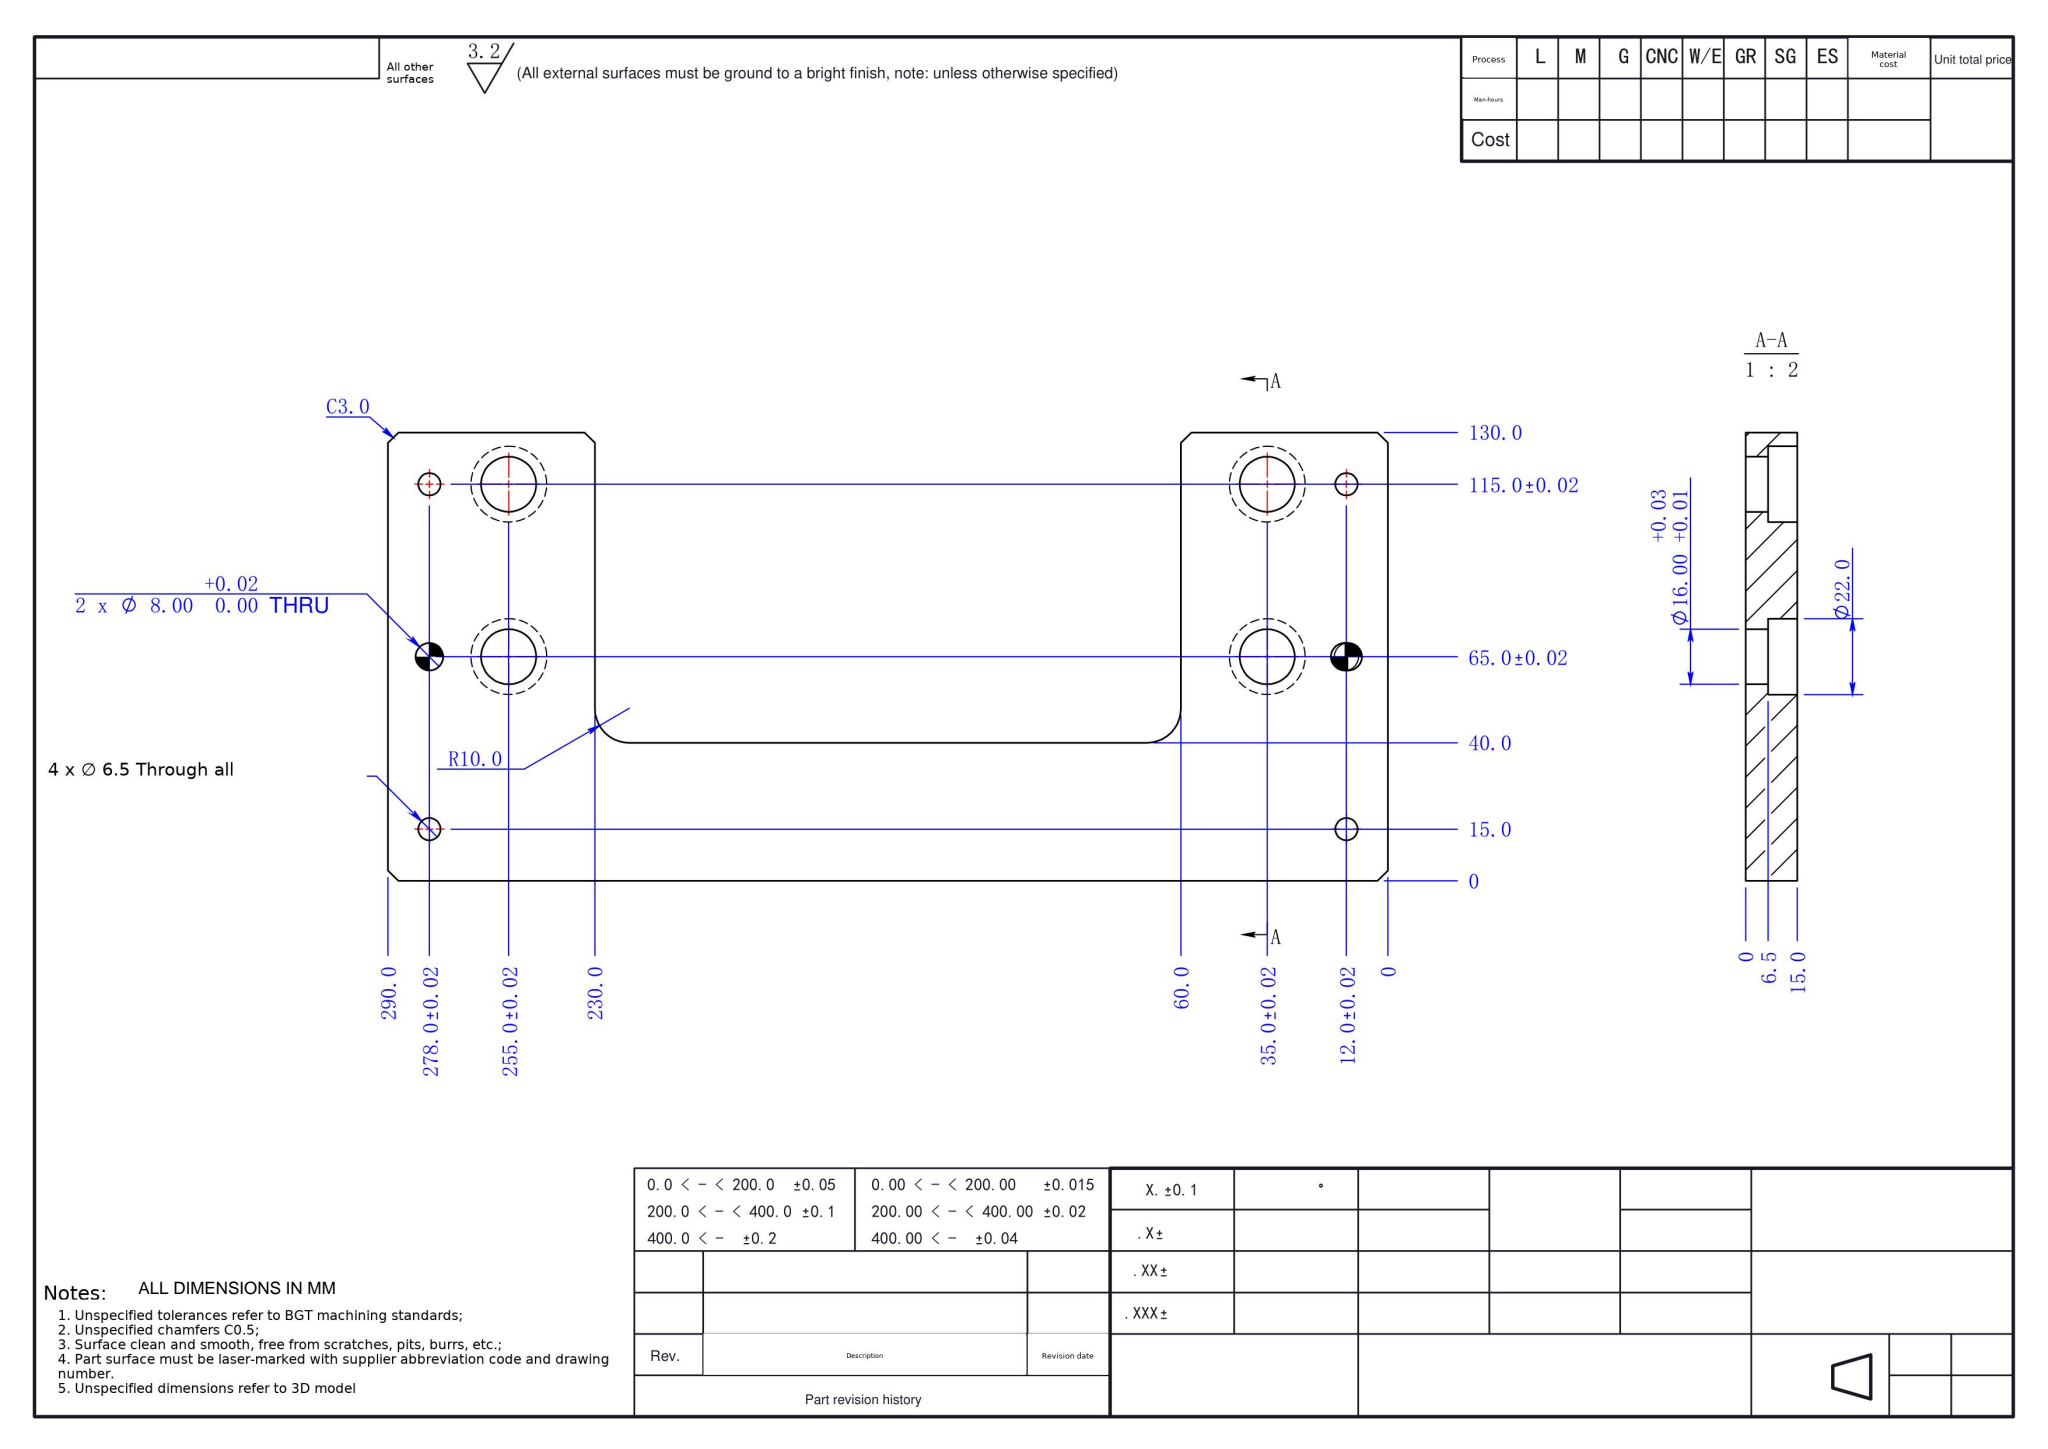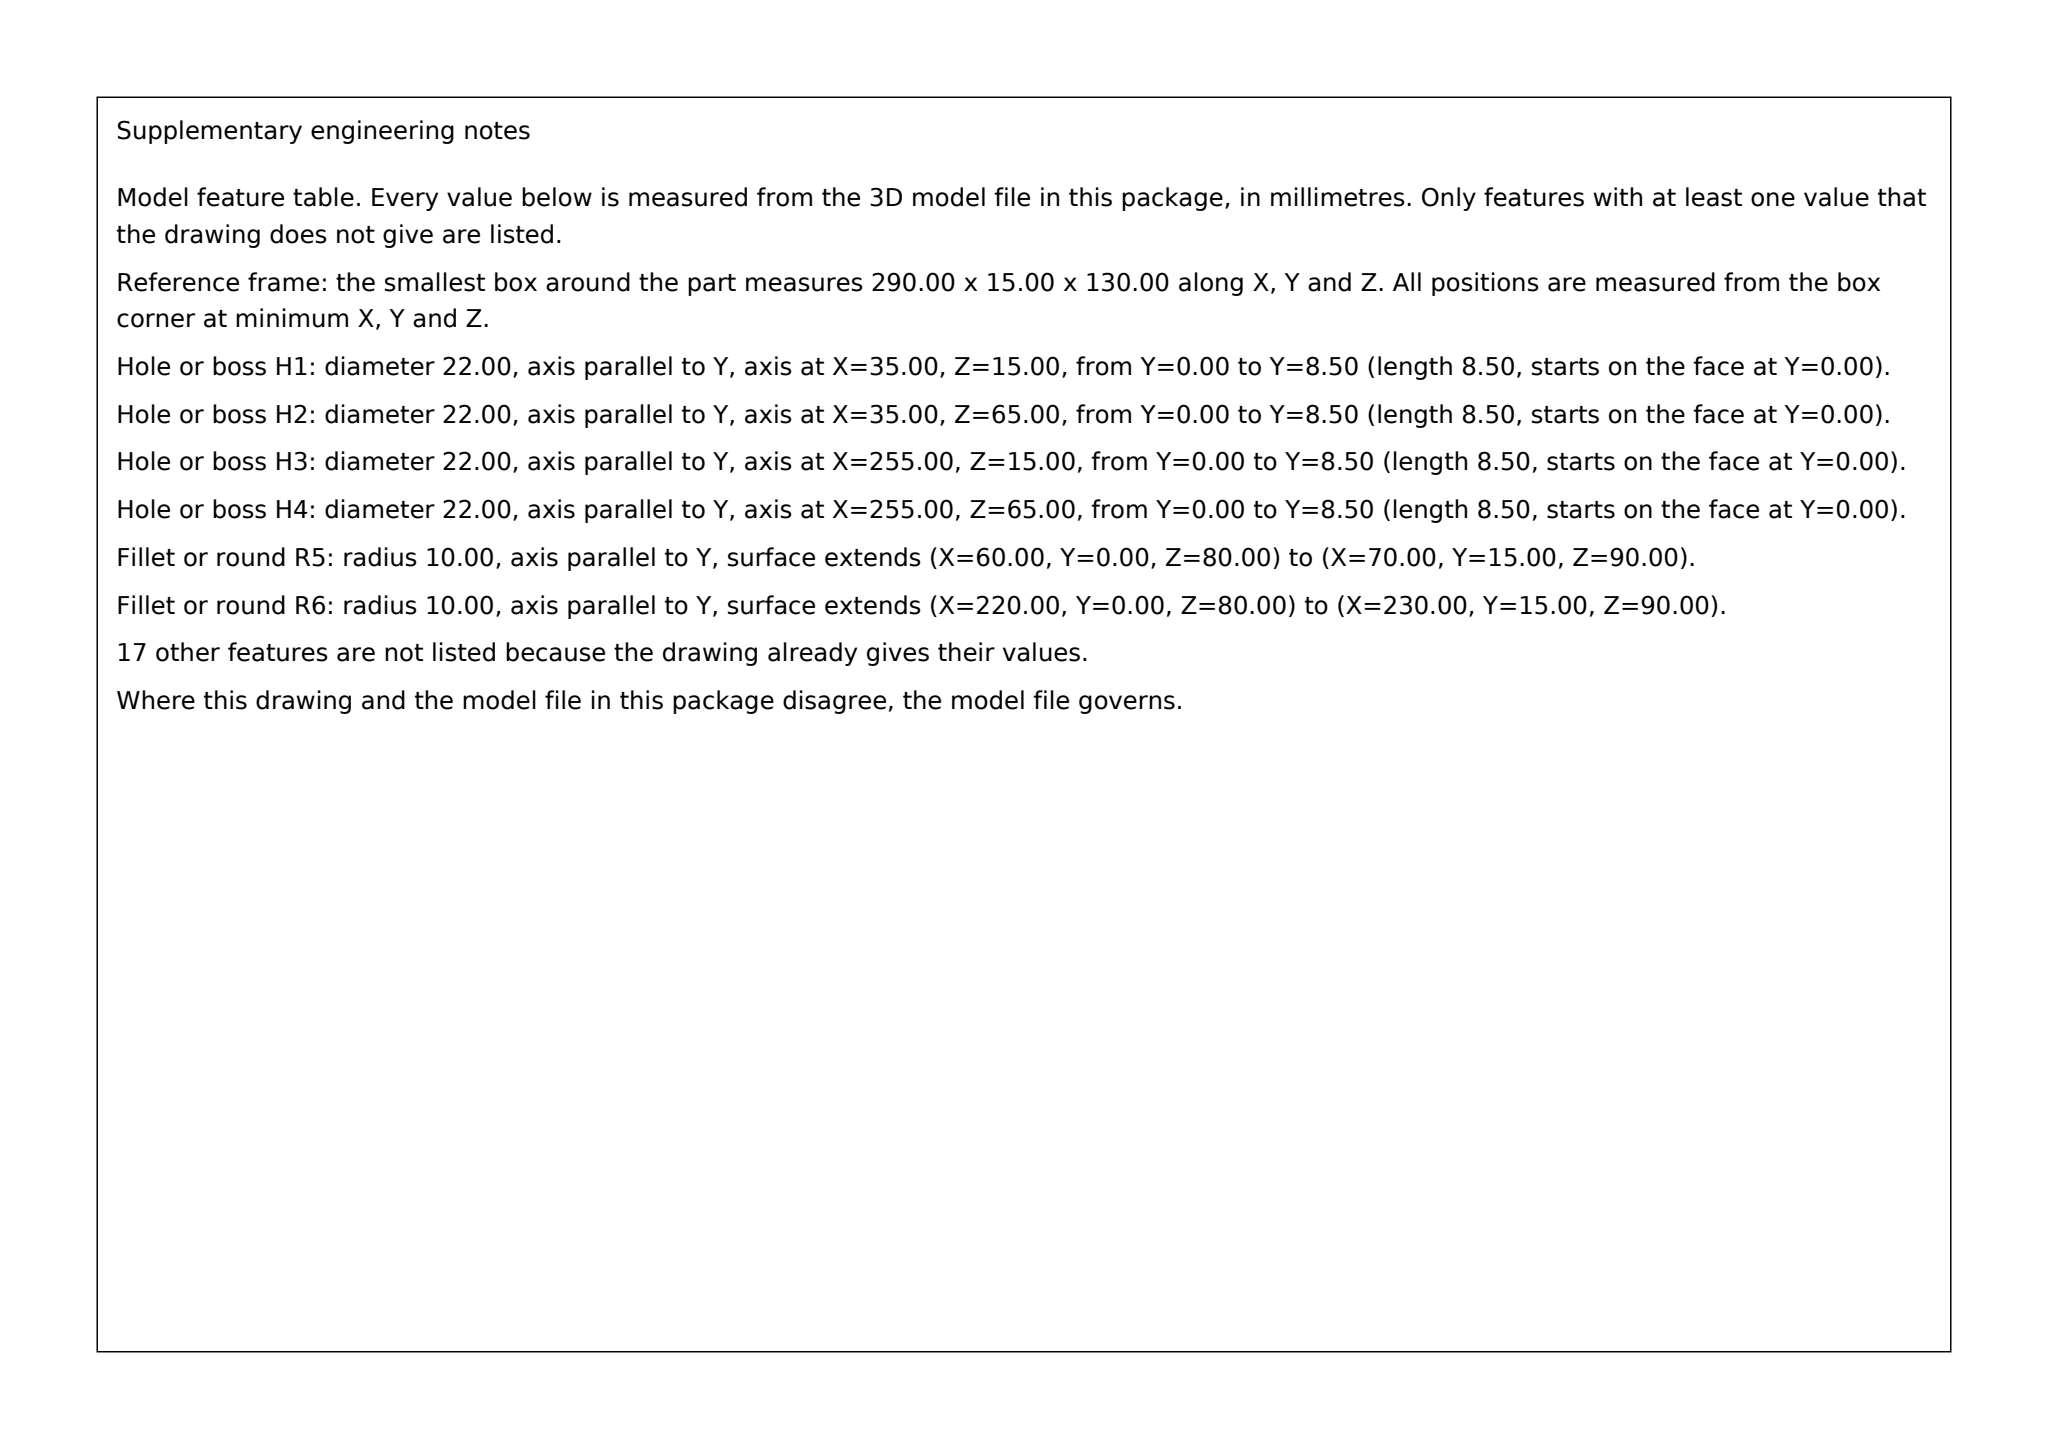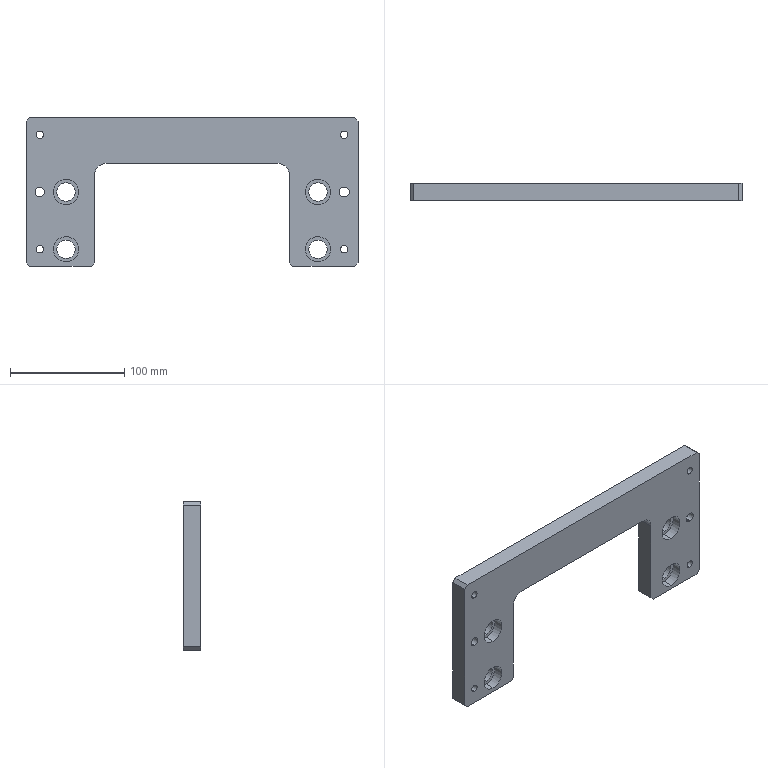Part | SolidWorks | mm | 1 solid | 52 faces | box 290 x 15 x 130 mm | volume 314468 mm3 | cylinder 30 | plane 22 | commonest cylinder face diameters 6.5 x8 22 x8 16 x8 8 x4 20 x2
build123d program:
from build123d import *

# Parameters (mm, degrees)
SKETCH1_W                  = 250
SKETCH1_H                  = 80
BOSS_EXTRUDE1_DEPTH        = 15
SKETCH13_R                 = 8
CUT_EXTRUDE4_DEPTH         = 133.098
SKETCH15_R                 = 11
CUT_EXTRUDE6_DEPTH         = 8.5
SKETCH18_W                 = 250
SKETCH18_H                 = 15
BOSS_EXTRUDE2_DEPTH        = 50
SKETCH20_W                 = 170
SKETCH20_H                 = 90
CUT_EXTRUDE9_DEPTH         = 155.758
FILLET1_R                  = 10
SKETCH21_W                 = 130
SKETCH21_H                 = 15
BOSS_EXTRUDE3_DEPTH        = 20
SKETCH22_W                 = 130
SKETCH22_H                 = 15
BOSS_EXTRUDE4_DEPTH        = 20
F_6_5_6_5_DIAMETER_HOLE1_D = 6.5
CHAMFER1_SIZE              = 3
SIZE_MM_DOWEL_PIN_HOLE1_D  = 8
CUT_EXTRUDE10_DEPTH        = 172.318


with BuildPart() as part:
    # Sketch1 → Boss-Extrude1 (new body)
    with BuildSketch(Plane(origin=(0, 0, 0), x_dir=(1, 0, 0), z_dir=(0, 1, 0))):
        Rectangle(SKETCH1_W, SKETCH1_H)
    extrude(amount=BOSS_EXTRUDE1_DEPTH)

    # Sketch13 → Cut-Extrude4 (cut, through all)
    with BuildSketch(Plane(origin=(0, 15, 0), x_dir=(1, 0, 0), z_dir=(0, 1, 0))):
        with Locations(Location((110, 25, 0), (0, 0, 270))):
            Circle(SKETCH13_R)
        with Locations(Location((-110, 25, 0), (0, 0, 90))):
            Circle(SKETCH13_R)
        with Locations(Location((-110, -25, 0), (0, 0, 270))):
            Circle(SKETCH13_R)
        with Locations(Location((110, -25, 0), (0, 0, 90))):
            Circle(SKETCH13_R)
    extrude(amount=-CUT_EXTRUDE4_DEPTH, mode=Mode.SUBTRACT)

    # Sketch15 → Cut-Extrude6 (cut)
    with BuildSketch(Plane.XZ):
        with Locations(Location((110, 25, 0), (0, 0, 270))):
            Circle(SKETCH15_R)
        with Locations(Location((110, -25, 0), (0, 0, 270))):
            Circle(SKETCH15_R)
        with Locations(Location((-110, -25, 0), (0, 0, 270))):
            Circle(SKETCH15_R)
        with Locations(Location((-110, 25, 0), (0, 0, 270))):
            Circle(SKETCH15_R)
    extrude(amount=-CUT_EXTRUDE6_DEPTH, mode=Mode.SUBTRACT)

    # Sketch18 → Boss-Extrude2 (add)
    with BuildSketch(Plane.XY.offset(40)):
        with Locations((0, 7.5)):
            Rectangle(SKETCH18_W, SKETCH18_H)
    extrude(amount=BOSS_EXTRUDE2_DEPTH)

    # Sketch20 → Cut-Extrude9 (cut, through all)
    with BuildSketch(Plane.XZ):
        with Locations((0, 5)):
            Rectangle(SKETCH20_W, SKETCH20_H)
    extrude(amount=-CUT_EXTRUDE9_DEPTH, mode=Mode.SUBTRACT)

    # Fillet1
    fillet1_edges = [part.edges().sort_by_distance(p)[0] for p in [
        (-85, 7.5, 50),
        (85, 7.5, 50),
    ]]
    fillet(fillet1_edges, radius=FILLET1_R)

    # Sketch21 → Boss-Extrude3 (add)
    with BuildSketch(Plane(origin=(125, 0, 0), x_dir=(0, 0, -1), z_dir=(1, 0, 0))):
        with Locations((-25, 7.5)):
            Rectangle(SKETCH21_W, SKETCH21_H)
    extrude(amount=BOSS_EXTRUDE3_DEPTH)

    # Sketch22 → Boss-Extrude4 (add)
    with BuildSketch(Plane.ZY.offset(125)):
        with Locations((25, 7.5)):
            Rectangle(SKETCH22_W, SKETCH22_H)
    extrude(amount=BOSS_EXTRUDE4_DEPTH)

    # 6.5 _6.5_ Diameter Hole1 (through all)
    with Locations(Plane(origin=(0, 15, 0), x_dir=(1, 0, 0), z_dir=(0, 1, 0))):
        with Locations((-133, 25), (-133, -75), (133, -75), (133, 25)):
            Hole(F_6_5_6_5_DIAMETER_HOLE1_D / 2)

    # Chamfer1
    chamfer1_edges = [part.edges().sort_by_distance(p)[0] for p in [
        (-145, 7.5, -40),
        (-145, 7.5, 90),
        (-85, 7.5, -40),
        (85, 7.5, -40),
        (145, 7.5, 90),
        (145, 7.5, -40),
    ]]
    chamfer(chamfer1_edges, length=CHAMFER1_SIZE)

    # Size mm Dowel Pin Hole1 (through all)
    with Locations(Plane(origin=(0, 15, 0), x_dir=(1, 0, 0), z_dir=(0, 1, 0))):
        with Locations((-133, -25), (133, -25)):
            Hole(SIZE_MM_DOWEL_PIN_HOLE1_D / 2)

    # Sketch27 → Cut-Extrude10 (cut, through all)
    with BuildSketch(Plane.XZ):
        with BuildLine():
            Line((132.5, 29), (133.5, 29))
            ThreePointArc((133.5, 29), (137.5, 25), (133.5, 21))
            Line((133.5, 21), (132.5, 21))
            ThreePointArc((132.5, 21), (128.5, 25), (132.5, 29))
        make_face()
    extrude(amount=-CUT_EXTRUDE10_DEPTH, mode=Mode.SUBTRACT)


solid = part.part